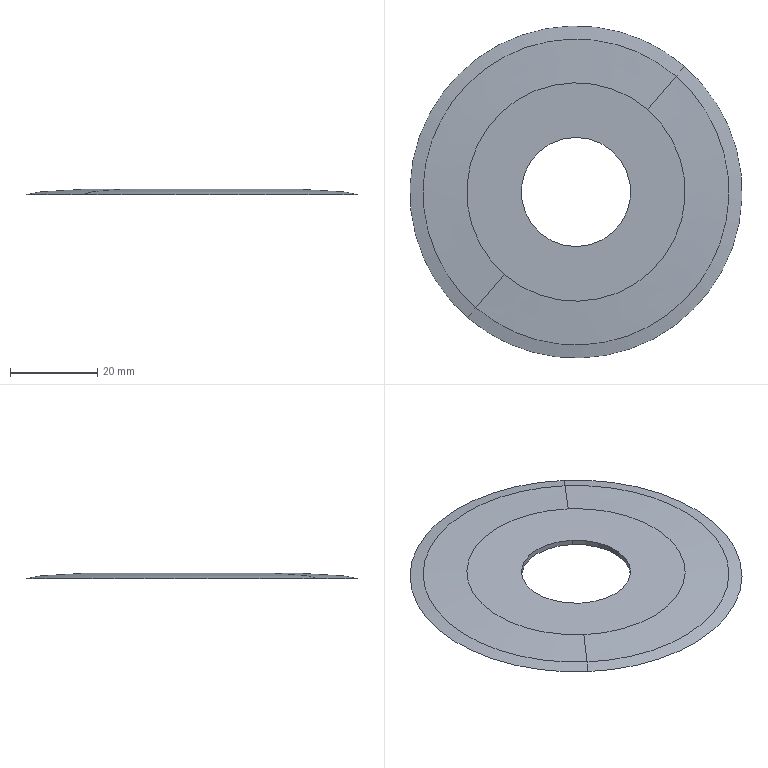Component | SolidWorks | 108SingleEdgeBlade0-23 | 1 solid | 8 faces | box 76 x 76 x 1.2 mm | volume 3636 mm3 | cone 4 | cylinder 2 | plane 2 | commonest cylinder face diameters 25 x2
build123d program:
from build123d import *

# Parameters (mm, degrees)
SKETCH3_R          = 12.5
CUT_EXTRUDE2_DEPTH = 10


with BuildPart() as part:
    # Sketch1 → Revolve1 (revolve)
    with BuildSketch(Plane(origin=(0, 0, 0), x_dir=(0, 0, -1), z_dir=(1, 0, 0)), mode=Mode.PRIVATE) as revolve1_sk:
        Polygon((-0.6, 5), (-0.6, 38), (0, 35), (0.6, 25), (0.6, 5), align=None)
    revolve(revolve1_sk.sketch.rotate(Axis((0, 0, 5.329), (0, 0, -1)), 90), axis=Axis((0, 0, 5.329), (0, 0, -1)))

    # Sketch3 → Cut-Extrude2 (cut)
    with BuildSketch(Plane(origin=(0, 0, -0.6), x_dir=(-1, 0, 0), z_dir=(0, 0, -1))):
        Circle(SKETCH3_R)
    extrude(amount=-CUT_EXTRUDE2_DEPTH, mode=Mode.SUBTRACT)


solid = part.part

# Placed as in the assembly
solid = solid.moved(Location((-15.093, -37.782, 222.855), (180, 0, 0)))
STEP:
#1=CARTESIAN_POINT('',(-0.9164,-1.859,8.75));
#2=VERTEX_POINT('',#1);
#3=CARTESIAN_POINT('',(-0.2721,-1.115,8.75));
#4=VERTEX_POINT('',#3);
#5=CARTESIAN_POINT('',(-0.5942,-1.487,8.75));
#6=DIRECTION('',(0.,-0.,1.));
#7=DIRECTION('',(0.6546,0.756,0.));
#8=AXIS2_PLACEMENT_3D('',#5,#6,#7);
#9=CIRCLE('',#8,0.4921);
#10=EDGE_CURVE('',#2,#4,#9,.T.);
#11=ORIENTED_EDGE('',*,*,#10,.F.);
#12=CARTESIAN_POINT('',(-0.9164,-1.859,8.797));
#13=VERTEX_POINT('',#12);
#14=CARTESIAN_POINT('',(-0.9164,-1.859,8.404));
#15=DIRECTION('',(0.,-0.,1.));
#16=VECTOR('',#15,39.37);
#17=LINE('',#14,#16);
#18=EDGE_CURVE('',#2,#13,#17,.T.);
#19=ORIENTED_EDGE('',*,*,#18,.T.);
#20=CARTESIAN_POINT('',(-0.2721,-1.115,8.797));
#21=VERTEX_POINT('',#20);
#22=CARTESIAN_POINT('',(-0.5942,-1.487,8.797));
#23=DIRECTION('',(0.,-0.,1.));
#24=DIRECTION('',(0.6546,0.756,0.));
#25=AXIS2_PLACEMENT_3D('',#22,#23,#24);
#26=CIRCLE('',#25,0.4921);
#27=EDGE_CURVE('',#13,#21,#26,.T.);
#28=ORIENTED_EDGE('',*,*,#27,.T.);
#29=CARTESIAN_POINT('',(-0.2721,-1.115,8.404));
#30=DIRECTION('',(0.,-0.,1.));
#31=VECTOR('',#30,39.37);
#32=LINE('',#29,#31);
#33=EDGE_CURVE('',#4,#21,#32,.T.);
#34=ORIENTED_EDGE('',*,*,#33,.F.);
#35=EDGE_LOOP('',(#11,#19,#28,#34));
#36=FACE_OUTER_BOUND('',#35,.T.);
#37=CARTESIAN_POINT('',(-0.5942,-1.487,8.404));
#38=DIRECTION('',(0.,-0.,1.));
#39=DIRECTION('',(0.6546,0.756,0.));
#40=AXIS2_PLACEMENT_3D('',#37,#38,#39);
#41=CYLINDRICAL_SURFACE('',#40,0.4921);
#42=ADVANCED_FACE('',(#36),#41,.F.);
#43=CARTESIAN_POINT('',(-1.239,-2.232,8.797));
#44=VERTEX_POINT('',#43);
#45=CARTESIAN_POINT('',(0.0501,-0.7434,8.797));
#46=VERTEX_POINT('',#45);
#47=CARTESIAN_POINT('',(-0.5942,-1.487,8.797));
#48=DIRECTION('',(-0.,0.,-1.));
#49=DIRECTION('',(-0.6546,-0.756,0.));
#50=AXIS2_PLACEMENT_3D('',#47,#48,#49);
#51=CIRCLE('',#50,0.9843);
#52=EDGE_CURVE('',#44,#46,#51,.T.);
#53=ORIENTED_EDGE('',*,*,#52,.T.);
#54=CARTESIAN_POINT('',(0.3078,-0.4458,8.774));
#55=VERTEX_POINT('',#54);
#56=CARTESIAN_POINT('',(0.0501,-0.7434,8.797));
#57=DIRECTION('',(0.6535,0.7546,-0.05989));
#58=VECTOR('',#57,39.37);
#59=LINE('',#56,#58);
#60=EDGE_CURVE('',#46,#55,#59,.T.);
#61=ORIENTED_EDGE('',*,*,#60,.T.);
#62=CARTESIAN_POINT('',(-1.496,-2.529,8.774));
#63=VERTEX_POINT('',#62);
#64=CARTESIAN_POINT('',(-0.5942,-1.487,8.774));
#65=DIRECTION('',(-0.,0.,-1.));
#66=DIRECTION('',(-0.6546,-0.756,0.));
#67=AXIS2_PLACEMENT_3D('',#64,#65,#66);
#68=CIRCLE('',#67,1.378);
#69=EDGE_CURVE('',#63,#55,#68,.T.);
#70=ORIENTED_EDGE('',*,*,#69,.F.);
#71=CARTESIAN_POINT('',(-1.239,-2.232,8.797));
#72=DIRECTION('',(-0.6535,-0.7546,-0.05989));
#73=VECTOR('',#72,39.37);
#74=LINE('',#71,#73);
#75=EDGE_CURVE('',#44,#63,#74,.T.);
#76=ORIENTED_EDGE('',*,*,#75,.F.);
#77=EDGE_LOOP('',(#53,#61,#70,#76));
#78=FACE_OUTER_BOUND('',#77,.T.);
#79=CARTESIAN_POINT('',(-0.5942,-1.487,8.797));
#80=DIRECTION('',(-0.,0.,-1.));
#81=DIRECTION('',(-0.6546,-0.756,0.));
#82=AXIS2_PLACEMENT_3D('',#79,#80,#81);
#83=CONICAL_SURFACE('',#82,0.9843,1.511);
#84=ADVANCED_FACE('',(#78),#83,.T.);
#85=ORIENTED_EDGE('',*,*,#69,.T.);
#86=CARTESIAN_POINT('',(0.3851,-0.3565,8.75));
#87=VERTEX_POINT('',#86);
#88=CARTESIAN_POINT('',(0.3078,-0.4458,8.774));
#89=DIRECTION('',(0.6419,0.7413,-0.1961));
#90=VECTOR('',#89,39.37);
#91=LINE('',#88,#90);
#92=EDGE_CURVE('',#55,#87,#91,.T.);
#93=ORIENTED_EDGE('',*,*,#92,.T.);
#94=CARTESIAN_POINT('',(-1.574,-2.618,8.75));
#95=VERTEX_POINT('',#94);
#96=CARTESIAN_POINT('',(-0.5942,-1.487,8.75));
#97=DIRECTION('',(-0.,0.,-1.));
#98=DIRECTION('',(-0.6546,-0.756,0.));
#99=AXIS2_PLACEMENT_3D('',#96,#97,#98);
#100=CIRCLE('',#99,1.496);
#101=EDGE_CURVE('',#95,#87,#100,.T.);
#102=ORIENTED_EDGE('',*,*,#101,.F.);
#103=CARTESIAN_POINT('',(-1.496,-2.529,8.774));
#104=DIRECTION('',(-0.6419,-0.7413,-0.1961));
#105=VECTOR('',#104,39.37);
#106=LINE('',#103,#105);
#107=EDGE_CURVE('',#63,#95,#106,.T.);
#108=ORIENTED_EDGE('',*,*,#107,.F.);
#109=EDGE_LOOP('',(#85,#93,#102,#108));
#110=FACE_OUTER_BOUND('',#109,.T.);
#111=CARTESIAN_POINT('',(-0.5942,-1.487,8.774));
#112=DIRECTION('',(-0.,0.,-1.));
#113=DIRECTION('',(-0.6546,-0.756,0.));
#114=AXIS2_PLACEMENT_3D('',#111,#112,#113);
#115=CONICAL_SURFACE('',#114,1.378,1.373);
#116=ADVANCED_FACE('',(#110),#115,.T.);
#117=CARTESIAN_POINT('',(-0.5942,-1.487,8.75));
#118=DIRECTION('',(0.,-0.,1.));
#119=DIRECTION('',(0.6546,0.756,0.));
#120=AXIS2_PLACEMENT_3D('',#117,#118,#119);
#121=CIRCLE('',#120,0.4921);
#122=EDGE_CURVE('',#4,#2,#121,.T.);
#123=ORIENTED_EDGE('',*,*,#122,.T.);
#124=ORIENTED_EDGE('',*,*,#10,.T.);
#125=EDGE_LOOP('',(#123,#124));
#126=FACE_BOUND('',#125,.T.);
#127=ORIENTED_EDGE('',*,*,#101,.T.);
#128=CARTESIAN_POINT('',(-0.5942,-1.487,8.75));
#129=DIRECTION('',(-0.,0.,-1.));
#130=DIRECTION('',(-0.6546,-0.756,0.));
#131=AXIS2_PLACEMENT_3D('',#128,#129,#130);
#132=CIRCLE('',#131,1.496);
#133=EDGE_CURVE('',#87,#95,#132,.T.);
#134=ORIENTED_EDGE('',*,*,#133,.T.);
#135=EDGE_LOOP('',(#127,#134));
#136=FACE_OUTER_BOUND('',#135,.T.);
#137=CARTESIAN_POINT('',(-0.743,-1.359,8.75));
#138=DIRECTION('',(0.,-0.,1.));
#139=DIRECTION('',(0.6546,0.756,0.));
#140=AXIS2_PLACEMENT_3D('',#137,#138,#139);
#141=PLANE('',#140);
#142=ADVANCED_FACE('',(#126,#136),#141,.F.);
#143=ORIENTED_EDGE('',*,*,#92,.F.);
#144=CARTESIAN_POINT('',(-0.5942,-1.487,8.774));
#145=DIRECTION('',(-0.,0.,-1.));
#146=DIRECTION('',(-0.6546,-0.756,0.));
#147=AXIS2_PLACEMENT_3D('',#144,#145,#146);
#148=CIRCLE('',#147,1.378);
#149=EDGE_CURVE('',#55,#63,#148,.T.);
#150=ORIENTED_EDGE('',*,*,#149,.T.);
#151=ORIENTED_EDGE('',*,*,#107,.T.);
#152=ORIENTED_EDGE('',*,*,#133,.F.);
#153=EDGE_LOOP('',(#143,#150,#151,#152));
#154=FACE_OUTER_BOUND('',#153,.T.);
#155=CARTESIAN_POINT('',(-0.5942,-1.487,8.774));
#156=DIRECTION('',(-0.,0.,-1.));
#157=DIRECTION('',(-0.6546,-0.756,0.));
#158=AXIS2_PLACEMENT_3D('',#155,#156,#157);
#159=CONICAL_SURFACE('',#158,1.378,1.373);
#160=ADVANCED_FACE('',(#154),#159,.T.);
#161=ORIENTED_EDGE('',*,*,#60,.F.);
#162=CARTESIAN_POINT('',(-0.5942,-1.487,8.797));
#163=DIRECTION('',(-0.,0.,-1.));
#164=DIRECTION('',(-0.6546,-0.756,0.));
#165=AXIS2_PLACEMENT_3D('',#162,#163,#164);
#166=CIRCLE('',#165,0.9843);
#167=EDGE_CURVE('',#46,#44,#166,.T.);
#168=ORIENTED_EDGE('',*,*,#167,.T.);
#169=ORIENTED_EDGE('',*,*,#75,.T.);
#170=ORIENTED_EDGE('',*,*,#149,.F.);
#171=EDGE_LOOP('',(#161,#168,#169,#170));
#172=FACE_OUTER_BOUND('',#171,.T.);
#173=CARTESIAN_POINT('',(-0.5942,-1.487,8.797));
#174=DIRECTION('',(-0.,0.,-1.));
#175=DIRECTION('',(-0.6546,-0.756,0.));
#176=AXIS2_PLACEMENT_3D('',#173,#174,#175);
#177=CONICAL_SURFACE('',#176,0.9843,1.511);
#178=ADVANCED_FACE('',(#172),#177,.T.);
#179=CARTESIAN_POINT('',(-0.5942,-1.487,8.797));
#180=DIRECTION('',(0.,-0.,1.));
#181=DIRECTION('',(0.6546,0.756,0.));
#182=AXIS2_PLACEMENT_3D('',#179,#180,#181);
#183=CIRCLE('',#182,0.4921);
#184=EDGE_CURVE('',#21,#13,#183,.T.);
#185=ORIENTED_EDGE('',*,*,#184,.F.);
#186=ORIENTED_EDGE('',*,*,#27,.F.);
#187=EDGE_LOOP('',(#185,#186));
#188=FACE_BOUND('',#187,.T.);
#189=ORIENTED_EDGE('',*,*,#52,.F.);
#190=ORIENTED_EDGE('',*,*,#167,.F.);
#191=EDGE_LOOP('',(#189,#190));
#192=FACE_OUTER_BOUND('',#191,.T.);
#193=CARTESIAN_POINT('',(-1.338,-0.8431,8.797));
#194=DIRECTION('',(-0.,0.,-1.));
#195=DIRECTION('',(-0.6546,-0.756,-0.));
#196=AXIS2_PLACEMENT_3D('',#193,#194,#195);
#197=PLANE('',#196);
#198=ADVANCED_FACE('',(#188,#192),#197,.F.);
#199=ORIENTED_EDGE('',*,*,#18,.F.);
#200=ORIENTED_EDGE('',*,*,#122,.F.);
#201=ORIENTED_EDGE('',*,*,#33,.T.);
#202=ORIENTED_EDGE('',*,*,#184,.T.);
#203=EDGE_LOOP('',(#199,#200,#201,#202));
#204=FACE_OUTER_BOUND('',#203,.T.);
#205=CARTESIAN_POINT('',(-0.5942,-1.487,8.404));
#206=DIRECTION('',(0.,-0.,1.));
#207=DIRECTION('',(0.6546,0.756,0.));
#208=AXIS2_PLACEMENT_3D('',#205,#206,#207);
#209=CYLINDRICAL_SURFACE('',#208,0.4921);
#210=ADVANCED_FACE('',(#204),#209,.F.);
#211=CLOSED_SHELL('',(#42,#84,#116,#142,#160,#178,#198,#210));
#212=MANIFOLD_SOLID_BREP('',#211);
#213=CARTESIAN_POINT('',(0.,0.,0.));
#214=DIRECTION('',(0.,0.,1.));
#215=DIRECTION('',(1.,0.,0.));
#216=AXIS2_PLACEMENT_3D('',#213,#214,#215);
#217=(LENGTH_UNIT()NAMED_UNIT(*)SI_UNIT($,.METRE.));
#218=LENGTH_MEASURE_WITH_UNIT(LENGTH_MEASURE(0.0254),#217);
#219=DIMENSIONAL_EXPONENTS(1.,0.,0.,0.,0.,0.,0.);
#220=(CONVERSION_BASED_UNIT('',#218)LENGTH_UNIT()NAMED_UNIT(#219));
#221=UNCERTAINTY_MEASURE_WITH_UNIT(LENGTH_MEASURE(0.00001),#220,'','');
#222=(NAMED_UNIT(*)PLANE_ANGLE_UNIT()SI_UNIT($,.RADIAN.));
#223=(NAMED_UNIT(*)SI_UNIT($,.STERADIAN.)SOLID_ANGLE_UNIT());
#224=(GEOMETRIC_REPRESENTATION_CONTEXT(3)GLOBAL_UNCERTAINTY_ASSIGNED_CONTEXT((#221))GLOBAL_UNIT_ASSIGNED_CONTEXT((#220,#222,#223))REPRESENTATION_CONTEXT('',''));
#225=ADVANCED_BREP_SHAPE_REPRESENTATION('',(#212,#216),#224);
#226=COLOUR_RGB('',0.7922,0.8196,0.9333);
#227=FILL_AREA_STYLE_COLOUR('',#226);
#228=FILL_AREA_STYLE('',(#227));
#229=SURFACE_STYLE_FILL_AREA(#228);
#230=SURFACE_SIDE_STYLE('',(#229));
#231=SURFACE_STYLE_USAGE(.BOTH.,#230);
#232=PRESENTATION_STYLE_ASSIGNMENT((#231));
#233=STYLED_ITEM('',(#232),#212);
#234=PRESENTATION_LAYER_ASSIGNMENT('','',(#233));
#235=(LENGTH_UNIT()NAMED_UNIT(*)SI_UNIT($,.METRE.));
#236=LENGTH_MEASURE_WITH_UNIT(LENGTH_MEASURE(0.0254),#235);
#237=DIMENSIONAL_EXPONENTS(1.,0.,0.,0.,0.,0.,0.);
#238=(CONVERSION_BASED_UNIT('',#236)LENGTH_UNIT()NAMED_UNIT(#237));
#239=UNCERTAINTY_MEASURE_WITH_UNIT(LENGTH_MEASURE(0.00001),#238,'','');
#240=(NAMED_UNIT(*)PLANE_ANGLE_UNIT()SI_UNIT($,.RADIAN.));
#241=(NAMED_UNIT(*)SI_UNIT($,.STERADIAN.)SOLID_ANGLE_UNIT());
#242=(GEOMETRIC_REPRESENTATION_CONTEXT(3)GLOBAL_UNCERTAINTY_ASSIGNED_CONTEXT((#239))GLOBAL_UNIT_ASSIGNED_CONTEXT((#238,#240,#241))REPRESENTATION_CONTEXT('',''));
#243=MECHANICAL_DESIGN_GEOMETRIC_PRESENTATION_REPRESENTATION('',(#233),#242);